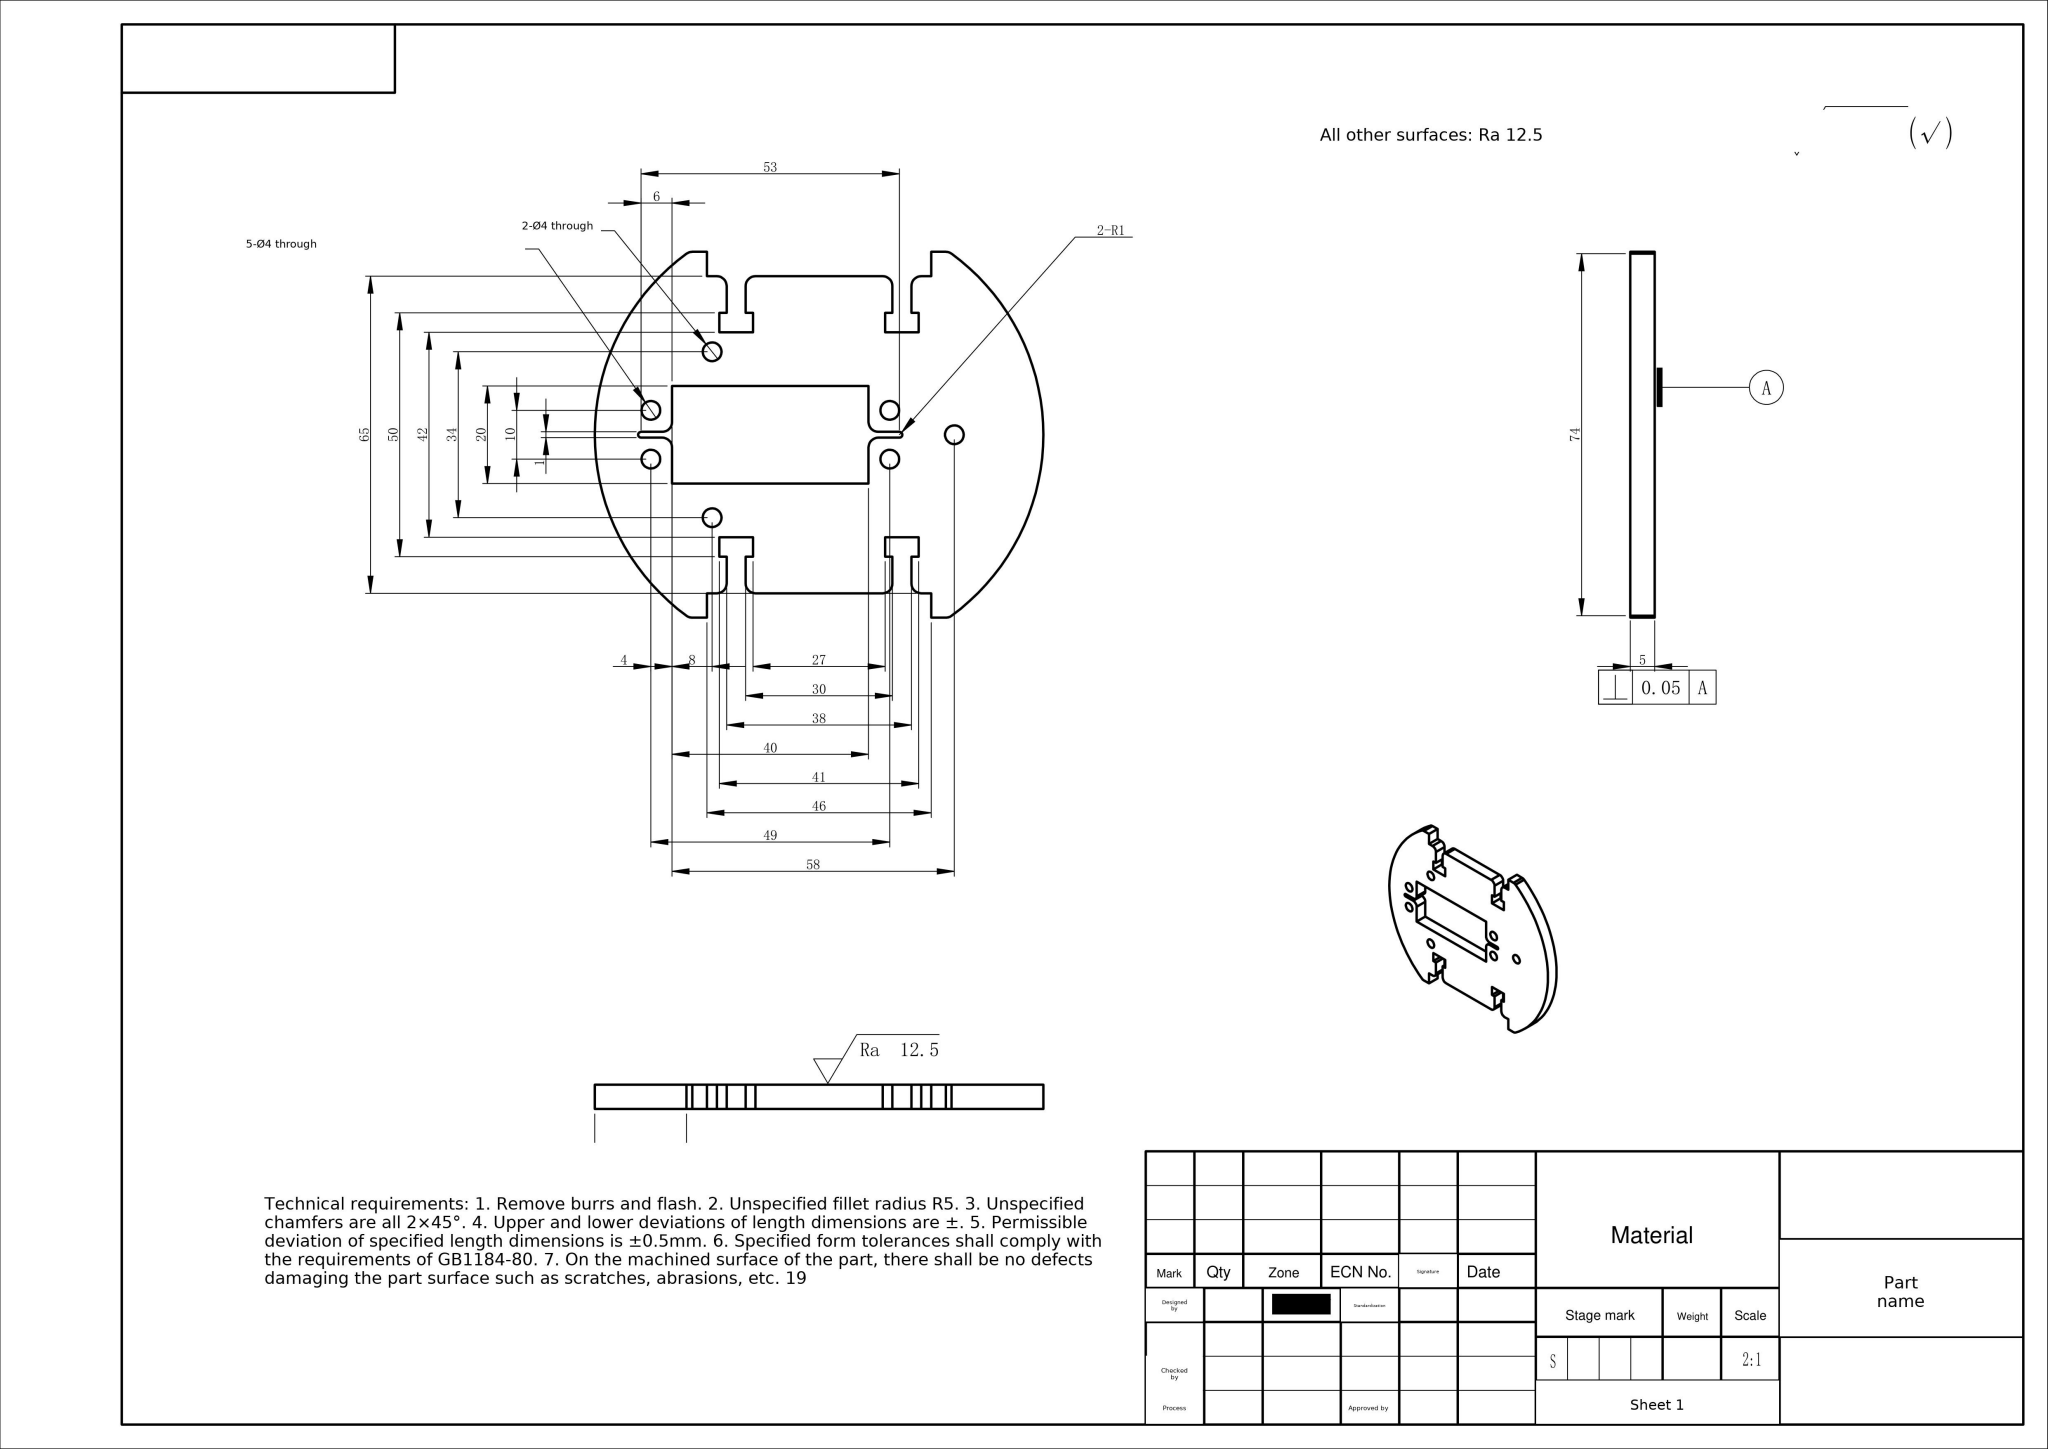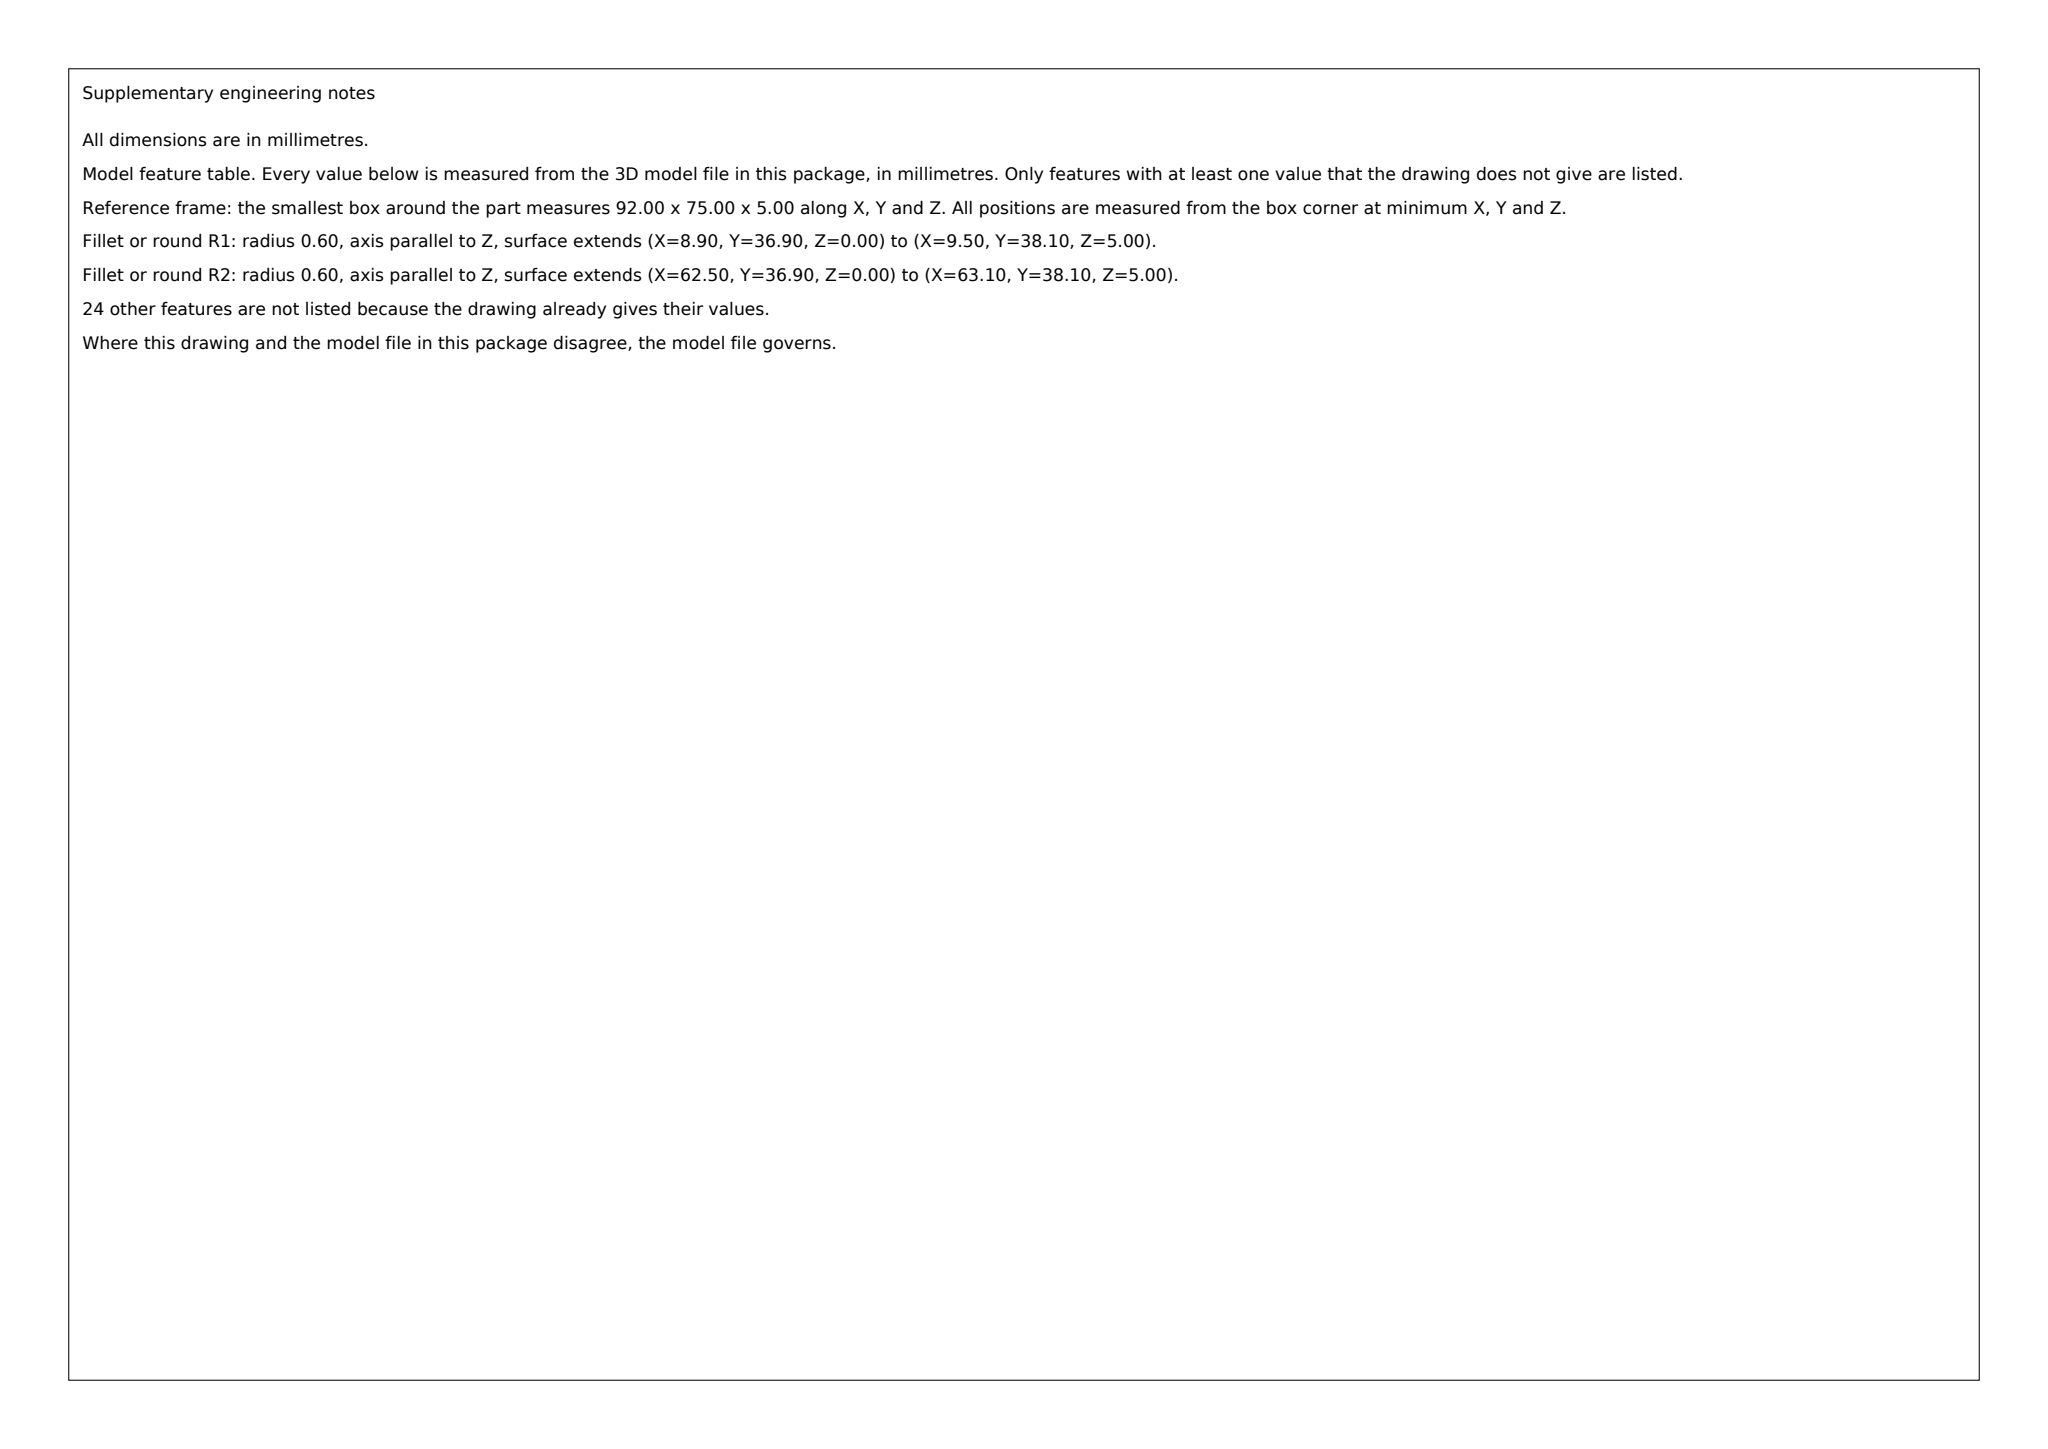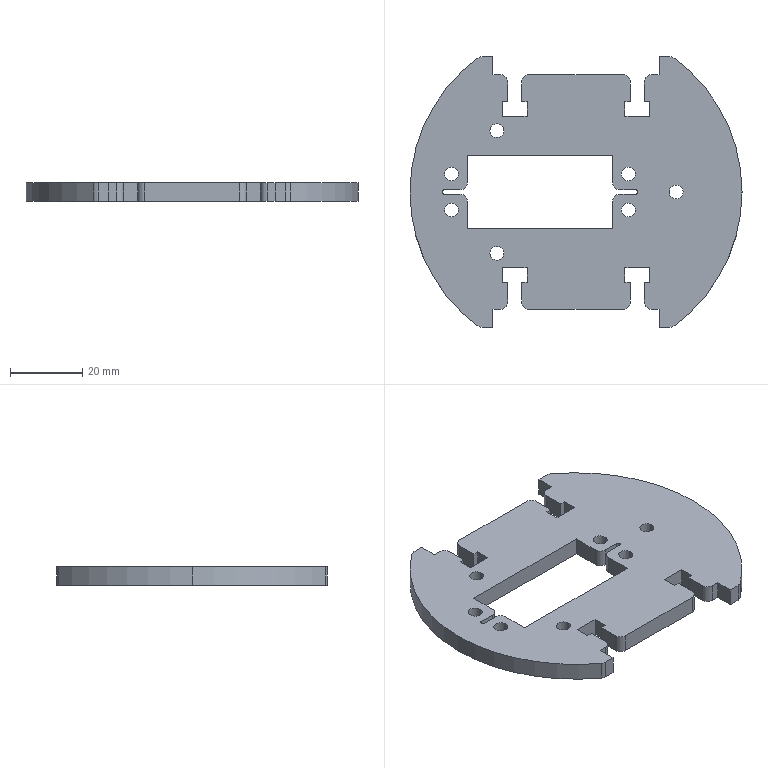Part | SolidWorks | mm | 1 solid | 90 faces | box 92 x 75 x 5 mm | volume 22149 mm3 | plane 54 | cylinder 36 | commonest cylinder face diameters 4 x16 3.85 x14 1.2 x3 92 x3
build123d program:
from build123d import *

# Parameters (mm, degrees)
ESQUISSE1_R        = 1.925
BOSS_EXTRU_1_DEPTH = 5


with BuildPart() as part:
    # Esquisse1 → Boss.-Extru.1 (new body)
    with BuildSketch(Plane.XY):
        with BuildLine():
            Line((13.05, 32.5), (-13.05, 32.5))
            ThreePointArc((-13.05, 32.5), (-14.464, 31.914), (-15.05, 30.5))
            Line((-15.05, 30.5), (-15.05, 25))
            Line((-15.05, 25), (-13.55, 25))
            Line((-13.55, 25), (-13.55, 21))
            Line((-13.55, 21), (-20.45, 21))
            Line((-20.45, 21), (-20.45, 25))
            Line((-20.45, 25), (-18.95, 25))
            Line((-18.95, 25), (-18.95, 30.5))
            ThreePointArc((-18.95, 30.5), (-19.536, 31.914), (-20.95, 32.5))
            Line((-20.95, 32.5), (-23, 32.5))
            Line((-23, 32.5), (-23, 37.5))
            Line((-23, 37.5), (-26, 37.498))
            ThreePointArc((-26, 37.498), (-26.621, 37.398), (-27.18, 37.111))
            ThreePointArc((-27.18, 37.111), (-46, 0), (-27.18, -37.111))
            ThreePointArc((-27.18, -37.111), (-26.621, -37.398), (-26, -37.498))
            Line((-26, -37.498), (-23, -37.5))
            Line((-23, -37.5), (-23, -32.5))
            Line((-23, -32.5), (-20.95, -32.5))
            ThreePointArc((-20.95, -32.5), (-19.536, -31.914), (-18.95, -30.5))
            Line((-18.95, -30.5), (-18.95, -25))
            Line((-18.95, -25), (-20.45, -25))
            Line((-20.45, -25), (-20.45, -21))
            Line((-20.45, -21), (-13.55, -21))
            Line((-13.55, -21), (-13.55, -25))
            Line((-13.55, -25), (-15.05, -25))
            Line((-15.05, -25), (-15.05, -30.5))
            ThreePointArc((-15.05, -30.5), (-14.464, -31.914), (-13.05, -32.5))
            Line((-13.05, -32.5), (13.05, -32.5))
            ThreePointArc((13.05, -32.5), (14.464, -31.914), (15.05, -30.5))
            Line((15.05, -30.5), (15.05, -25))
            Line((15.05, -25), (13.55, -25))
            Line((13.55, -25), (13.55, -21))
            Line((13.55, -21), (20.45, -21))
            Line((20.45, -21), (20.45, -25))
            Line((20.45, -25), (18.95, -25))
            Line((18.95, -25), (18.95, -30.5))
            ThreePointArc((18.95, -30.5), (19.536, -31.914), (20.95, -32.5))
            Line((20.95, -32.5), (23, -32.5))
            Line((23, -32.5), (23, -37.5))
            Line((23, -37.5), (26, -37.498))
            ThreePointArc((26, -37.498), (26.621, -37.398), (27.18, -37.111))
            ThreePointArc((27.18, -37.111), (46, 0), (27.18, 37.111))
            ThreePointArc((27.18, 37.111), (26.621, 37.398), (26, 37.498))
            Line((26, 37.498), (23, 37.5))
            Line((23, 37.5), (23, 32.5))
            Line((23, 32.5), (20.95, 32.5))
            ThreePointArc((20.95, 32.5), (19.536, 31.914), (18.95, 30.5))
            Line((18.95, 30.5), (18.95, 25))
            Line((18.95, 25), (20.45, 25))
            Line((20.45, 25), (20.45, 21))
            Line((20.45, 21), (13.55, 21))
            Line((13.55, 21), (13.55, 25))
            Line((13.55, 25), (15.05, 25))
            Line((15.05, 25), (15.05, 30.5))
            ThreePointArc((15.05, 30.5), (14.464, 31.914), (13.05, 32.5))
        make_face()
        with Locations((27.75, 0)):
            Circle(ESQUISSE1_R, mode=Mode.SUBTRACT)
        with Locations((-21.933, -17)):
            Circle(ESQUISSE1_R, mode=Mode.SUBTRACT)
        with Locations((-21.933, 17)):
            Circle(ESQUISSE1_R, mode=Mode.SUBTRACT)
        with Locations((14.5, -5)):
            Circle(ESQUISSE1_R, mode=Mode.SUBTRACT)
        with Locations((14.5, 5)):
            Circle(ESQUISSE1_R, mode=Mode.SUBTRACT)
        with Locations((-34.5, -5)):
            Circle(ESQUISSE1_R, mode=Mode.SUBTRACT)
        with Locations((-34.5, 5)):
            Circle(ESQUISSE1_R, mode=Mode.SUBTRACT)
        with BuildLine():
            Line((10.15, -10), (10.15, -2.6))
            ThreePointArc((10.15, -2.6), (10.736, -1.186), (12.15, -0.6))
            Line((12.15, -0.6), (16.5, -0.6))
            ThreePointArc((16.5, -0.6), (17.1, 0), (16.5, 0.6))
            Line((16.5, 0.6), (12.15, 0.6))
            ThreePointArc((12.15, 0.6), (10.736, 1.186), (10.15, 2.6))
            Line((10.15, 2.6), (10.15, 10))
            Line((10.15, 10), (-30.15, 10))
            Line((-30.15, 10), (-30.15, 2.6))
            ThreePointArc((-30.15, 2.6), (-30.736, 1.186), (-32.15, 0.6))
            Line((-32.15, 0.6), (-36.5, 0.6))
            ThreePointArc((-36.5, 0.6), (-37.1, 0), (-36.5, -0.6))
            Line((-36.5, -0.6), (-32.15, -0.6))
            ThreePointArc((-32.15, -0.6), (-30.736, -1.186), (-30.15, -2.6))
            Line((-30.15, -2.6), (-30.15, -10))
            Line((-30.15, -10), (10.15, -10))
        make_face(mode=Mode.SUBTRACT)
    extrude(amount=BOSS_EXTRU_1_DEPTH)


solid = part.part